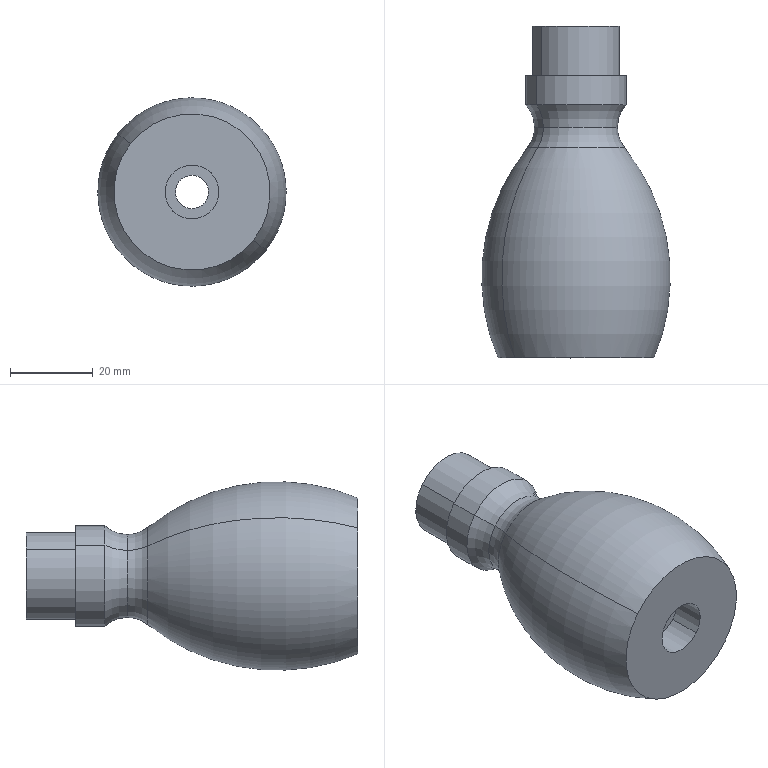Component | SolidWorks | 7-1 | 1 solid | 18 faces | volume 71833 mm3 | cylinder 8 | torus 6 | plane 4 | commonest cylinder face diameters 13 x2 8 x2 21 x2 24.16 x2
build123d program:
from build123d import *


with BuildPart() as part:
    # Sketch1 → Revolve1 (revolve)
    with BuildSketch(Plane.XY, mode=Mode.PRIVATE) as revolve1_sk:
        with BuildLine():
            Line((0, 10.5), (0, 4))
            Line((0, 4), (72, 4))
            Line((72, 4), (72, 6.5))
            Line((72, 6.5), (80, 6.5))
            Line((80, 6.5), (80, 18.83))
            ThreePointArc((80, 18.83), (53.719, 22.249), (29.382, 11.756))
            ThreePointArc((29.382, 11.756), (24.131, 10.004), (19, 12.08))
            Line((19, 12.08), (12, 12.08))
            Line((12, 12.08), (12, 10.5))
            Line((12, 10.5), (0, 10.5))
        make_face()
    revolve(revolve1_sk.sketch.rotate(Axis((0, 0, 0), (1, 0, 0)), 90), axis=Axis((0, 0, 0), (1, 0, 0)))


solid = part.part

# Placed as in the assembly
solid = solid.moved(Location((-132.516, 214.991, 571.696), (0, 0, -90)))
STEP:
#1=COLOUR_RGB('',0.7922,0.8196,0.9333);
#2=FILL_AREA_STYLE_COLOUR('',#1);
#3=FILL_AREA_STYLE('',(#2));
#4=SURFACE_STYLE_FILL_AREA(#3);
#5=SURFACE_SIDE_STYLE('',(#4));
#6=SURFACE_STYLE_USAGE(.BOTH.,#5);
#7=PRESENTATION_STYLE_ASSIGNMENT((#6));
#8=CARTESIAN_POINT('',(-5.591,7.716,22.801));
#9=VERTEX_POINT('',#8);
#10=CARTESIAN_POINT('',(-5.527,7.504,22.751));
#11=VERTEX_POINT('',#10);
#12=CARTESIAN_POINT('',(-5.774,7.504,22.945));
#13=DIRECTION('',(-0.6177,-0.,-0.7864));
#14=DIRECTION('',(-0.7864,0.,0.6177));
#15=AXIS2_PLACEMENT_3D('',#12,#13,#14);
#16=CIRCLE('',#15,0.315);
#17=EDGE_CURVE('',#9,#11,#16,.T.);
#18=ORIENTED_EDGE('',*,*,#17,.T.);
#19=CARTESIAN_POINT('',(-4.908,7.504,22.265));
#20=VERTEX_POINT('',#19);
#21=CARTESIAN_POINT('',(-5.217,7.504,22.508));
#22=DIRECTION('',(-0.,1.,-0.));
#23=DIRECTION('',(0.,0.,1.));
#24=AXIS2_PLACEMENT_3D('',#21,#22,#23);
#25=CIRCLE('',#24,0.3937);
#26=EDGE_CURVE('',#11,#20,#25,.T.);
#27=ORIENTED_EDGE('',*,*,#26,.T.);
#28=CARTESIAN_POINT('',(-4.843,7.716,22.214));
#29=VERTEX_POINT('',#28);
#30=CARTESIAN_POINT('',(-4.66,7.504,22.07));
#31=DIRECTION('',(0.6177,0.,0.7864));
#32=DIRECTION('',(0.7864,0.,-0.6177));
#33=AXIS2_PLACEMENT_3D('',#30,#31,#32);
#34=CIRCLE('',#33,0.315);
#35=EDGE_CURVE('',#29,#20,#34,.T.);
#36=ORIENTED_EDGE('',*,*,#35,.F.);
#37=CARTESIAN_POINT('',(-5.217,7.716,22.508));
#38=DIRECTION('',(-0.,1.,-0.));
#39=DIRECTION('',(-0.7864,0.,0.6177));
#40=AXIS2_PLACEMENT_3D('',#37,#38,#39);
#41=CIRCLE('',#40,0.4756);
#42=EDGE_CURVE('',#9,#29,#41,.T.);
#43=ORIENTED_EDGE('',*,*,#42,.F.);
#44=EDGE_LOOP('',(#18,#27,#36,#43));
#45=FACE_OUTER_BOUND('',#44,.T.);
#46=CARTESIAN_POINT('',(-5.217,7.504,22.508));
#47=DIRECTION('',(-0.,1.,-0.));
#48=DIRECTION('',(-0.7864,0.,0.6177));
#49=AXIS2_PLACEMENT_3D('',#46,#47,#48);
#50=TOROIDAL_SURFACE('',#49,0.7087,0.315);
#51=ADVANCED_FACE('',(#45),#50,.F.);
#52=ORIENTED_EDGE('',*,*,#35,.T.);
#53=CARTESIAN_POINT('',(-5.217,7.504,22.508));
#54=DIRECTION('',(-0.,1.,-0.));
#55=DIRECTION('',(0.,0.,1.));
#56=AXIS2_PLACEMENT_3D('',#53,#54,#55);
#57=CIRCLE('',#56,0.3937);
#58=EDGE_CURVE('',#20,#11,#57,.T.);
#59=ORIENTED_EDGE('',*,*,#58,.T.);
#60=ORIENTED_EDGE('',*,*,#17,.F.);
#61=CARTESIAN_POINT('',(-5.217,7.716,22.508));
#62=DIRECTION('',(-0.,1.,-0.));
#63=DIRECTION('',(-0.7864,0.,0.6177));
#64=AXIS2_PLACEMENT_3D('',#61,#62,#63);
#65=CIRCLE('',#64,0.4756);
#66=EDGE_CURVE('',#29,#9,#65,.T.);
#67=ORIENTED_EDGE('',*,*,#66,.F.);
#68=EDGE_LOOP('',(#52,#59,#60,#67));
#69=FACE_OUTER_BOUND('',#68,.T.);
#70=CARTESIAN_POINT('',(-5.217,7.504,22.508));
#71=DIRECTION('',(-0.,1.,-0.));
#72=DIRECTION('',(-0.7864,0.,0.6177));
#73=AXIS2_PLACEMENT_3D('',#70,#71,#72);
#74=TOROIDAL_SURFACE('',#73,0.7087,0.315);
#75=ADVANCED_FACE('',(#69),#74,.F.);
#76=CARTESIAN_POINT('',(-5.016,5.315,22.35));
#77=VERTEX_POINT('',#76);
#78=CARTESIAN_POINT('',(-5.418,5.315,22.666));
#79=VERTEX_POINT('',#78);
#80=CARTESIAN_POINT('',(-5.217,5.315,22.508));
#81=DIRECTION('',(-0.,1.,-0.));
#82=DIRECTION('',(-0.7864,0.,0.6177));
#83=AXIS2_PLACEMENT_3D('',#80,#81,#82);
#84=CIRCLE('',#83,0.2559);
#85=EDGE_CURVE('',#77,#79,#84,.T.);
#86=ORIENTED_EDGE('',*,*,#85,.F.);
#87=CARTESIAN_POINT('',(-5.016,5.63,22.35));
#88=VERTEX_POINT('',#87);
#89=CARTESIAN_POINT('',(-5.016,8.464,22.35));
#90=DIRECTION('',(-0.,1.,-0.));
#91=VECTOR('',#90,39.37);
#92=LINE('',#89,#91);
#93=EDGE_CURVE('',#77,#88,#92,.T.);
#94=ORIENTED_EDGE('',*,*,#93,.T.);
#95=CARTESIAN_POINT('',(-5.418,5.63,22.666));
#96=VERTEX_POINT('',#95);
#97=CARTESIAN_POINT('',(-5.217,5.63,22.508));
#98=DIRECTION('',(-0.,1.,-0.));
#99=DIRECTION('',(-0.7864,0.,0.6177));
#100=AXIS2_PLACEMENT_3D('',#97,#98,#99);
#101=CIRCLE('',#100,0.2559);
#102=EDGE_CURVE('',#88,#96,#101,.T.);
#103=ORIENTED_EDGE('',*,*,#102,.T.);
#104=CARTESIAN_POINT('',(-5.418,8.464,22.666));
#105=DIRECTION('',(-0.,1.,-0.));
#106=VECTOR('',#105,39.37);
#107=LINE('',#104,#106);
#108=EDGE_CURVE('',#79,#96,#107,.T.);
#109=ORIENTED_EDGE('',*,*,#108,.F.);
#110=EDGE_LOOP('',(#86,#94,#103,#109));
#111=FACE_OUTER_BOUND('',#110,.T.);
#112=CARTESIAN_POINT('',(-5.217,8.464,22.508));
#113=DIRECTION('',(-0.,1.,-0.));
#114=DIRECTION('',(-0.7864,0.,0.6177));
#115=AXIS2_PLACEMENT_3D('',#112,#113,#114);
#116=CYLINDRICAL_SURFACE('',#115,0.2559);
#117=ADVANCED_FACE('',(#111),#116,.F.);
#118=CARTESIAN_POINT('',(-5.093,5.63,22.41));
#119=VERTEX_POINT('',#118);
#120=CARTESIAN_POINT('',(-5.341,5.63,22.605));
#121=VERTEX_POINT('',#120);
#122=CARTESIAN_POINT('',(-5.217,5.63,22.508));
#123=DIRECTION('',(-0.,1.,-0.));
#124=DIRECTION('',(-0.7864,0.,0.6177));
#125=AXIS2_PLACEMENT_3D('',#122,#123,#124);
#126=CIRCLE('',#125,0.1575);
#127=EDGE_CURVE('',#119,#121,#126,.T.);
#128=ORIENTED_EDGE('',*,*,#127,.F.);
#129=CARTESIAN_POINT('',(-5.093,8.464,22.41));
#130=VERTEX_POINT('',#129);
#131=CARTESIAN_POINT('',(-5.093,8.464,22.41));
#132=DIRECTION('',(-0.,1.,-0.));
#133=VECTOR('',#132,39.37);
#134=LINE('',#131,#133);
#135=EDGE_CURVE('',#119,#130,#134,.T.);
#136=ORIENTED_EDGE('',*,*,#135,.T.);
#137=CARTESIAN_POINT('',(-5.341,8.464,22.605));
#138=VERTEX_POINT('',#137);
#139=CARTESIAN_POINT('',(-5.217,8.464,22.508));
#140=DIRECTION('',(-0.,1.,-0.));
#141=DIRECTION('',(-0.7864,0.,0.6177));
#142=AXIS2_PLACEMENT_3D('',#139,#140,#141);
#143=CIRCLE('',#142,0.1575);
#144=EDGE_CURVE('',#130,#138,#143,.T.);
#145=ORIENTED_EDGE('',*,*,#144,.T.);
#146=CARTESIAN_POINT('',(-5.341,8.464,22.605));
#147=DIRECTION('',(-0.,1.,-0.));
#148=VECTOR('',#147,39.37);
#149=LINE('',#146,#148);
#150=EDGE_CURVE('',#121,#138,#149,.T.);
#151=ORIENTED_EDGE('',*,*,#150,.F.);
#152=EDGE_LOOP('',(#128,#136,#145,#151));
#153=FACE_OUTER_BOUND('',#152,.T.);
#154=CARTESIAN_POINT('',(-5.217,8.464,22.508));
#155=DIRECTION('',(-0.,1.,-0.));
#156=DIRECTION('',(-0.7864,0.,0.6177));
#157=AXIS2_PLACEMENT_3D('',#154,#155,#156);
#158=CYLINDRICAL_SURFACE('',#157,0.1575);
#159=ADVANCED_FACE('',(#153),#158,.F.);
#160=CARTESIAN_POINT('',(-5.542,7.992,22.763));
#161=VERTEX_POINT('',#160);
#162=CARTESIAN_POINT('',(-4.892,7.992,22.252));
#163=VERTEX_POINT('',#162);
#164=CARTESIAN_POINT('',(-5.217,7.992,22.508));
#165=DIRECTION('',(-0.,1.,-0.));
#166=DIRECTION('',(-0.7864,0.,0.6177));
#167=AXIS2_PLACEMENT_3D('',#164,#165,#166);
#168=CIRCLE('',#167,0.4134);
#169=EDGE_CURVE('',#161,#163,#168,.T.);
#170=ORIENTED_EDGE('',*,*,#169,.T.);
#171=CARTESIAN_POINT('',(-4.892,8.464,22.252));
#172=VERTEX_POINT('',#171);
#173=CARTESIAN_POINT('',(-4.892,8.464,22.252));
#174=DIRECTION('',(-0.,1.,-0.));
#175=VECTOR('',#174,39.37);
#176=LINE('',#173,#175);
#177=EDGE_CURVE('',#163,#172,#176,.T.);
#178=ORIENTED_EDGE('',*,*,#177,.T.);
#179=CARTESIAN_POINT('',(-5.542,8.464,22.763));
#180=VERTEX_POINT('',#179);
#181=CARTESIAN_POINT('',(-5.217,8.464,22.508));
#182=DIRECTION('',(-0.,1.,-0.));
#183=DIRECTION('',(-0.7864,0.,0.6177));
#184=AXIS2_PLACEMENT_3D('',#181,#182,#183);
#185=CIRCLE('',#184,0.4134);
#186=EDGE_CURVE('',#180,#172,#185,.T.);
#187=ORIENTED_EDGE('',*,*,#186,.F.);
#188=CARTESIAN_POINT('',(-5.542,8.464,22.763));
#189=DIRECTION('',(-0.,1.,-0.));
#190=VECTOR('',#189,39.37);
#191=LINE('',#188,#190);
#192=EDGE_CURVE('',#161,#180,#191,.T.);
#193=ORIENTED_EDGE('',*,*,#192,.F.);
#194=EDGE_LOOP('',(#170,#178,#187,#193));
#195=FACE_OUTER_BOUND('',#194,.T.);
#196=CARTESIAN_POINT('',(-5.217,8.464,22.508));
#197=DIRECTION('',(-0.,1.,-0.));
#198=DIRECTION('',(-0.7864,0.,0.6177));
#199=AXIS2_PLACEMENT_3D('',#196,#197,#198);
#200=CYLINDRICAL_SURFACE('',#199,0.4134);
#201=ADVANCED_FACE('',(#195),#200,.T.);
#202=ORIENTED_EDGE('',*,*,#42,.T.);
#203=CARTESIAN_POINT('',(-4.843,7.992,22.214));
#204=VERTEX_POINT('',#203);
#205=CARTESIAN_POINT('',(-4.843,8.464,22.214));
#206=DIRECTION('',(-0.,1.,-0.));
#207=VECTOR('',#206,39.37);
#208=LINE('',#205,#207);
#209=EDGE_CURVE('',#29,#204,#208,.T.);
#210=ORIENTED_EDGE('',*,*,#209,.T.);
#211=CARTESIAN_POINT('',(-5.591,7.992,22.801));
#212=VERTEX_POINT('',#211);
#213=CARTESIAN_POINT('',(-5.217,7.992,22.508));
#214=DIRECTION('',(-0.,1.,-0.));
#215=DIRECTION('',(-0.7864,0.,0.6177));
#216=AXIS2_PLACEMENT_3D('',#213,#214,#215);
#217=CIRCLE('',#216,0.4756);
#218=EDGE_CURVE('',#212,#204,#217,.T.);
#219=ORIENTED_EDGE('',*,*,#218,.F.);
#220=CARTESIAN_POINT('',(-5.591,8.464,22.801));
#221=DIRECTION('',(-0.,1.,-0.));
#222=VECTOR('',#221,39.37);
#223=LINE('',#220,#222);
#224=EDGE_CURVE('',#9,#212,#223,.T.);
#225=ORIENTED_EDGE('',*,*,#224,.F.);
#226=EDGE_LOOP('',(#202,#210,#219,#225));
#227=FACE_OUTER_BOUND('',#226,.T.);
#228=CARTESIAN_POINT('',(-5.217,8.464,22.508));
#229=DIRECTION('',(-0.,1.,-0.));
#230=DIRECTION('',(-0.7864,0.,0.6177));
#231=AXIS2_PLACEMENT_3D('',#228,#229,#230);
#232=CYLINDRICAL_SURFACE('',#231,0.4756);
#233=ADVANCED_FACE('',(#227),#232,.T.);
#234=ORIENTED_EDGE('',*,*,#58,.F.);
#235=CARTESIAN_POINT('',(-4.853,7.307,22.222));
#236=VERTEX_POINT('',#235);
#237=CARTESIAN_POINT('',(-4.66,7.504,22.07));
#238=DIRECTION('',(0.6177,0.,0.7864));
#239=DIRECTION('',(0.7864,0.,-0.6177));
#240=AXIS2_PLACEMENT_3D('',#237,#238,#239);
#241=CIRCLE('',#240,0.315);
#242=EDGE_CURVE('',#20,#236,#241,.T.);
#243=ORIENTED_EDGE('',*,*,#242,.T.);
#244=CARTESIAN_POINT('',(-5.581,7.307,22.794));
#245=VERTEX_POINT('',#244);
#246=CARTESIAN_POINT('',(-5.217,7.307,22.508));
#247=DIRECTION('',(-0.,1.,-0.));
#248=DIRECTION('',(-0.7864,0.,0.6177));
#249=AXIS2_PLACEMENT_3D('',#246,#247,#248);
#250=CIRCLE('',#249,0.4628);
#251=EDGE_CURVE('',#236,#245,#250,.T.);
#252=ORIENTED_EDGE('',*,*,#251,.T.);
#253=CARTESIAN_POINT('',(-5.774,7.504,22.945));
#254=DIRECTION('',(-0.6177,-0.,-0.7864));
#255=DIRECTION('',(-0.7864,0.,0.6177));
#256=AXIS2_PLACEMENT_3D('',#253,#254,#255);
#257=CIRCLE('',#256,0.315);
#258=EDGE_CURVE('',#11,#245,#257,.T.);
#259=ORIENTED_EDGE('',*,*,#258,.F.);
#260=EDGE_LOOP('',(#234,#243,#252,#259));
#261=FACE_OUTER_BOUND('',#260,.T.);
#262=CARTESIAN_POINT('',(-5.217,7.504,22.508));
#263=DIRECTION('',(-0.,1.,-0.));
#264=DIRECTION('',(-0.7864,0.,0.6177));
#265=AXIS2_PLACEMENT_3D('',#262,#263,#264);
#266=TOROIDAL_SURFACE('',#265,0.7087,0.315);
#267=ADVANCED_FACE('',(#261),#266,.F.);
#268=CARTESIAN_POINT('',(-5.8,5.315,22.966));
#269=VERTEX_POINT('',#268);
#270=CARTESIAN_POINT('',(-4.634,5.315,22.05));
#271=VERTEX_POINT('',#270);
#272=CARTESIAN_POINT('',(-5.217,5.315,22.508));
#273=DIRECTION('',(-0.,1.,-0.));
#274=DIRECTION('',(-0.7864,0.,0.6177));
#275=AXIS2_PLACEMENT_3D('',#272,#273,#274);
#276=CIRCLE('',#275,0.7414);
#277=EDGE_CURVE('',#269,#271,#276,.T.);
#278=ORIENTED_EDGE('',*,*,#277,.T.);
#279=CARTESIAN_POINT('',(-6.061,6.077,23.171));
#280=DIRECTION('',(0.6177,0.,0.7864));
#281=DIRECTION('',(0.7864,0.,-0.6177));
#282=AXIS2_PLACEMENT_3D('',#279,#280,#281);
#283=CIRCLE('',#282,1.969);
#284=EDGE_CURVE('',#271,#236,#283,.T.);
#285=ORIENTED_EDGE('',*,*,#284,.T.);
#286=CARTESIAN_POINT('',(-5.217,7.307,22.508));
#287=DIRECTION('',(-0.,1.,-0.));
#288=DIRECTION('',(-0.7864,0.,0.6177));
#289=AXIS2_PLACEMENT_3D('',#286,#287,#288);
#290=CIRCLE('',#289,0.4628);
#291=EDGE_CURVE('',#245,#236,#290,.T.);
#292=ORIENTED_EDGE('',*,*,#291,.F.);
#293=CARTESIAN_POINT('',(-4.373,6.077,21.845));
#294=DIRECTION('',(-0.6177,-0.,-0.7864));
#295=DIRECTION('',(-0.7864,0.,0.6177));
#296=AXIS2_PLACEMENT_3D('',#293,#294,#295);
#297=CIRCLE('',#296,1.969);
#298=EDGE_CURVE('',#269,#245,#297,.T.);
#299=ORIENTED_EDGE('',*,*,#298,.F.);
#300=EDGE_LOOP('',(#278,#285,#292,#299));
#301=FACE_OUTER_BOUND('',#300,.T.);
#302=CARTESIAN_POINT('',(-5.217,6.077,22.508));
#303=DIRECTION('',(-0.,1.,-0.));
#304=DIRECTION('',(-0.7864,0.,0.6177));
#305=AXIS2_PLACEMENT_3D('',#302,#303,#304);
#306=TOROIDAL_SURFACE('',#305,-1.074,1.969);
#307=ADVANCED_FACE('',(#301),#306,.T.);
#308=ORIENTED_EDGE('',*,*,#284,.F.);
#309=CARTESIAN_POINT('',(-5.217,5.315,22.508));
#310=DIRECTION('',(-0.,1.,-0.));
#311=DIRECTION('',(-0.7864,0.,0.6177));
#312=AXIS2_PLACEMENT_3D('',#309,#310,#311);
#313=CIRCLE('',#312,0.7414);
#314=EDGE_CURVE('',#271,#269,#313,.T.);
#315=ORIENTED_EDGE('',*,*,#314,.T.);
#316=ORIENTED_EDGE('',*,*,#298,.T.);
#317=ORIENTED_EDGE('',*,*,#251,.F.);
#318=EDGE_LOOP('',(#308,#315,#316,#317));
#319=FACE_OUTER_BOUND('',#318,.T.);
#320=CARTESIAN_POINT('',(-5.217,6.077,22.508));
#321=DIRECTION('',(-0.,1.,-0.));
#322=DIRECTION('',(-0.7864,0.,0.6177));
#323=AXIS2_PLACEMENT_3D('',#320,#321,#322);
#324=TOROIDAL_SURFACE('',#323,-1.074,1.969);
#325=ADVANCED_FACE('',(#319),#324,.T.);
#326=ORIENTED_EDGE('',*,*,#26,.F.);
#327=ORIENTED_EDGE('',*,*,#258,.T.);
#328=ORIENTED_EDGE('',*,*,#291,.T.);
#329=ORIENTED_EDGE('',*,*,#242,.F.);
#330=EDGE_LOOP('',(#326,#327,#328,#329));
#331=FACE_OUTER_BOUND('',#330,.T.);
#332=CARTESIAN_POINT('',(-5.217,7.504,22.508));
#333=DIRECTION('',(-0.,1.,-0.));
#334=DIRECTION('',(-0.7864,0.,0.6177));
#335=AXIS2_PLACEMENT_3D('',#332,#333,#334);
#336=TOROIDAL_SURFACE('',#335,0.7087,0.315);
#337=ADVANCED_FACE('',(#331),#336,.F.);
#338=ORIENTED_EDGE('',*,*,#209,.F.);
#339=ORIENTED_EDGE('',*,*,#66,.T.);
#340=ORIENTED_EDGE('',*,*,#224,.T.);
#341=CARTESIAN_POINT('',(-5.217,7.992,22.508));
#342=DIRECTION('',(-0.,1.,-0.));
#343=DIRECTION('',(-0.7864,0.,0.6177));
#344=AXIS2_PLACEMENT_3D('',#341,#342,#343);
#345=CIRCLE('',#344,0.4756);
#346=EDGE_CURVE('',#204,#212,#345,.T.);
#347=ORIENTED_EDGE('',*,*,#346,.F.);
#348=EDGE_LOOP('',(#338,#339,#340,#347));
#349=FACE_OUTER_BOUND('',#348,.T.);
#350=CARTESIAN_POINT('',(-5.217,8.464,22.508));
#351=DIRECTION('',(-0.,1.,-0.));
#352=DIRECTION('',(-0.7864,0.,0.6177));
#353=AXIS2_PLACEMENT_3D('',#350,#351,#352);
#354=CYLINDRICAL_SURFACE('',#353,0.4756);
#355=ADVANCED_FACE('',(#349),#354,.T.);
#356=ORIENTED_EDGE('',*,*,#218,.T.);
#357=ORIENTED_EDGE('',*,*,#346,.T.);
#358=EDGE_LOOP('',(#356,#357));
#359=FACE_OUTER_BOUND('',#358,.T.);
#360=ORIENTED_EDGE('',*,*,#169,.F.);
#361=CARTESIAN_POINT('',(-5.217,7.992,22.508));
#362=DIRECTION('',(-0.,1.,-0.));
#363=DIRECTION('',(-0.7864,0.,0.6177));
#364=AXIS2_PLACEMENT_3D('',#361,#362,#363);
#365=CIRCLE('',#364,0.4134);
#366=EDGE_CURVE('',#163,#161,#365,.T.);
#367=ORIENTED_EDGE('',*,*,#366,.F.);
#368=EDGE_LOOP('',(#360,#367));
#369=FACE_BOUND('',#368,.T.);
#370=CARTESIAN_POINT('',(-5.217,7.992,22.508));
#371=DIRECTION('',(-0.,1.,-0.));
#372=DIRECTION('',(-0.7864,0.,0.6177));
#373=AXIS2_PLACEMENT_3D('',#370,#371,#372);
#374=PLANE('',#373);
#375=ADVANCED_FACE('',(#359,#369),#374,.T.);
#376=ORIENTED_EDGE('',*,*,#177,.F.);
#377=ORIENTED_EDGE('',*,*,#366,.T.);
#378=ORIENTED_EDGE('',*,*,#192,.T.);
#379=CARTESIAN_POINT('',(-5.217,8.464,22.508));
#380=DIRECTION('',(-0.,1.,-0.));
#381=DIRECTION('',(-0.7864,0.,0.6177));
#382=AXIS2_PLACEMENT_3D('',#379,#380,#381);
#383=CIRCLE('',#382,0.4134);
#384=EDGE_CURVE('',#172,#180,#383,.T.);
#385=ORIENTED_EDGE('',*,*,#384,.F.);
#386=EDGE_LOOP('',(#376,#377,#378,#385));
#387=FACE_OUTER_BOUND('',#386,.T.);
#388=CARTESIAN_POINT('',(-5.217,8.464,22.508));
#389=DIRECTION('',(-0.,1.,-0.));
#390=DIRECTION('',(-0.7864,0.,0.6177));
#391=AXIS2_PLACEMENT_3D('',#388,#389,#390);
#392=CYLINDRICAL_SURFACE('',#391,0.4134);
#393=ADVANCED_FACE('',(#387),#392,.T.);
#394=ORIENTED_EDGE('',*,*,#186,.T.);
#395=ORIENTED_EDGE('',*,*,#384,.T.);
#396=EDGE_LOOP('',(#394,#395));
#397=FACE_OUTER_BOUND('',#396,.T.);
#398=CARTESIAN_POINT('',(-5.217,8.464,22.508));
#399=DIRECTION('',(-0.,1.,-0.));
#400=DIRECTION('',(-0.7864,0.,0.6177));
#401=AXIS2_PLACEMENT_3D('',#398,#399,#400);
#402=CIRCLE('',#401,0.1575);
#403=EDGE_CURVE('',#138,#130,#402,.T.);
#404=ORIENTED_EDGE('',*,*,#403,.F.);
#405=ORIENTED_EDGE('',*,*,#144,.F.);
#406=EDGE_LOOP('',(#404,#405));
#407=FACE_BOUND('',#406,.T.);
#408=CARTESIAN_POINT('',(-5.217,8.464,22.508));
#409=DIRECTION('',(-0.,1.,-0.));
#410=DIRECTION('',(-0.7864,0.,0.6177));
#411=AXIS2_PLACEMENT_3D('',#408,#409,#410);
#412=PLANE('',#411);
#413=ADVANCED_FACE('',(#397,#407),#412,.T.);
#414=ORIENTED_EDGE('',*,*,#135,.F.);
#415=CARTESIAN_POINT('',(-5.217,5.63,22.508));
#416=DIRECTION('',(-0.,1.,-0.));
#417=DIRECTION('',(-0.7864,0.,0.6177));
#418=AXIS2_PLACEMENT_3D('',#415,#416,#417);
#419=CIRCLE('',#418,0.1575);
#420=EDGE_CURVE('',#121,#119,#419,.T.);
#421=ORIENTED_EDGE('',*,*,#420,.F.);
#422=ORIENTED_EDGE('',*,*,#150,.T.);
#423=ORIENTED_EDGE('',*,*,#403,.T.);
#424=EDGE_LOOP('',(#414,#421,#422,#423));
#425=FACE_OUTER_BOUND('',#424,.T.);
#426=CARTESIAN_POINT('',(-5.217,8.464,22.508));
#427=DIRECTION('',(-0.,1.,-0.));
#428=DIRECTION('',(-0.7864,0.,0.6177));
#429=AXIS2_PLACEMENT_3D('',#426,#427,#428);
#430=CYLINDRICAL_SURFACE('',#429,0.1575);
#431=ADVANCED_FACE('',(#425),#430,.F.);
#432=CARTESIAN_POINT('',(-5.217,5.63,22.508));
#433=DIRECTION('',(-0.,1.,-0.));
#434=DIRECTION('',(-0.7864,0.,0.6177));
#435=AXIS2_PLACEMENT_3D('',#432,#433,#434);
#436=CIRCLE('',#435,0.2559);
#437=EDGE_CURVE('',#96,#88,#436,.T.);
#438=ORIENTED_EDGE('',*,*,#437,.F.);
#439=ORIENTED_EDGE('',*,*,#102,.F.);
#440=EDGE_LOOP('',(#438,#439));
#441=FACE_OUTER_BOUND('',#440,.T.);
#442=ORIENTED_EDGE('',*,*,#420,.T.);
#443=ORIENTED_EDGE('',*,*,#127,.T.);
#444=EDGE_LOOP('',(#442,#443));
#445=FACE_BOUND('',#444,.T.);
#446=CARTESIAN_POINT('',(-5.217,5.63,22.508));
#447=DIRECTION('',(-0.,1.,-0.));
#448=DIRECTION('',(-0.7864,0.,0.6177));
#449=AXIS2_PLACEMENT_3D('',#446,#447,#448);
#450=PLANE('',#449);
#451=ADVANCED_FACE('',(#441,#445),#450,.F.);
#452=ORIENTED_EDGE('',*,*,#93,.F.);
#453=CARTESIAN_POINT('',(-5.217,5.315,22.508));
#454=DIRECTION('',(-0.,1.,-0.));
#455=DIRECTION('',(-0.7864,0.,0.6177));
#456=AXIS2_PLACEMENT_3D('',#453,#454,#455);
#457=CIRCLE('',#456,0.2559);
#458=EDGE_CURVE('',#79,#77,#457,.T.);
#459=ORIENTED_EDGE('',*,*,#458,.F.);
#460=ORIENTED_EDGE('',*,*,#108,.T.);
#461=ORIENTED_EDGE('',*,*,#437,.T.);
#462=EDGE_LOOP('',(#452,#459,#460,#461));
#463=FACE_OUTER_BOUND('',#462,.T.);
#464=CARTESIAN_POINT('',(-5.217,8.464,22.508));
#465=DIRECTION('',(-0.,1.,-0.));
#466=DIRECTION('',(-0.7864,0.,0.6177));
#467=AXIS2_PLACEMENT_3D('',#464,#465,#466);
#468=CYLINDRICAL_SURFACE('',#467,0.2559);
#469=ADVANCED_FACE('',(#463),#468,.F.);
#470=ORIENTED_EDGE('',*,*,#277,.F.);
#471=ORIENTED_EDGE('',*,*,#314,.F.);
#472=EDGE_LOOP('',(#470,#471));
#473=FACE_OUTER_BOUND('',#472,.T.);
#474=ORIENTED_EDGE('',*,*,#458,.T.);
#475=ORIENTED_EDGE('',*,*,#85,.T.);
#476=EDGE_LOOP('',(#474,#475));
#477=FACE_BOUND('',#476,.T.);
#478=CARTESIAN_POINT('',(-5.217,5.315,22.508));
#479=DIRECTION('',(-0.,1.,-0.));
#480=DIRECTION('',(-0.7864,0.,0.6177));
#481=AXIS2_PLACEMENT_3D('',#478,#479,#480);
#482=PLANE('',#481);
#483=ADVANCED_FACE('',(#473,#477),#482,.F.);
#484=CLOSED_SHELL('',(#51,#75,#117,#159,#201,#233,#267,#307,#325,#337,#355,#375,#393,#413,#431,#451,#469,#483));
#485=MANIFOLD_SOLID_BREP('',#484);
#486=STYLED_ITEM('',(#7),#485);
#487=(LENGTH_UNIT()NAMED_UNIT(*)SI_UNIT($,.METRE.));
#488=LENGTH_MEASURE_WITH_UNIT(LENGTH_MEASURE(0.0254),#487);
#489=DIMENSIONAL_EXPONENTS(1.,0.,0.,0.,0.,0.,0.);
#490=(CONVERSION_BASED_UNIT('',#488)LENGTH_UNIT()NAMED_UNIT(#489));
#491=UNCERTAINTY_MEASURE_WITH_UNIT(LENGTH_MEASURE(0.00001),#490,'','');
#492=(NAMED_UNIT(*)PLANE_ANGLE_UNIT()SI_UNIT($,.RADIAN.));
#493=(NAMED_UNIT(*)SI_UNIT($,.STERADIAN.)SOLID_ANGLE_UNIT());
#494=(GEOMETRIC_REPRESENTATION_CONTEXT(3)GLOBAL_UNCERTAINTY_ASSIGNED_CONTEXT((#491))GLOBAL_UNIT_ASSIGNED_CONTEXT((#490,#492,#493))REPRESENTATION_CONTEXT('',''));
#495=MECHANICAL_DESIGN_GEOMETRIC_PRESENTATION_REPRESENTATION('',(#486),#494);
#496=PRESENTATION_LAYER_ASSIGNMENT('','',(#486));
#497=CARTESIAN_POINT('',(0.,0.,0.));
#498=DIRECTION('',(0.,0.,1.));
#499=DIRECTION('',(1.,0.,0.));
#500=AXIS2_PLACEMENT_3D('',#497,#498,#499);
#501=(LENGTH_UNIT()NAMED_UNIT(*)SI_UNIT($,.METRE.));
#502=LENGTH_MEASURE_WITH_UNIT(LENGTH_MEASURE(0.0254),#501);
#503=DIMENSIONAL_EXPONENTS(1.,0.,0.,0.,0.,0.,0.);
#504=(CONVERSION_BASED_UNIT('',#502)LENGTH_UNIT()NAMED_UNIT(#503));
#505=UNCERTAINTY_MEASURE_WITH_UNIT(LENGTH_MEASURE(0.00001),#504,'','');
#506=(NAMED_UNIT(*)PLANE_ANGLE_UNIT()SI_UNIT($,.RADIAN.));
#507=(NAMED_UNIT(*)SI_UNIT($,.STERADIAN.)SOLID_ANGLE_UNIT());
#508=(GEOMETRIC_REPRESENTATION_CONTEXT(3)GLOBAL_UNCERTAINTY_ASSIGNED_CONTEXT((#505))GLOBAL_UNIT_ASSIGNED_CONTEXT((#504,#506,#507))REPRESENTATION_CONTEXT('',''));
#509=ADVANCED_BREP_SHAPE_REPRESENTATION('',(#485,#500),#508);